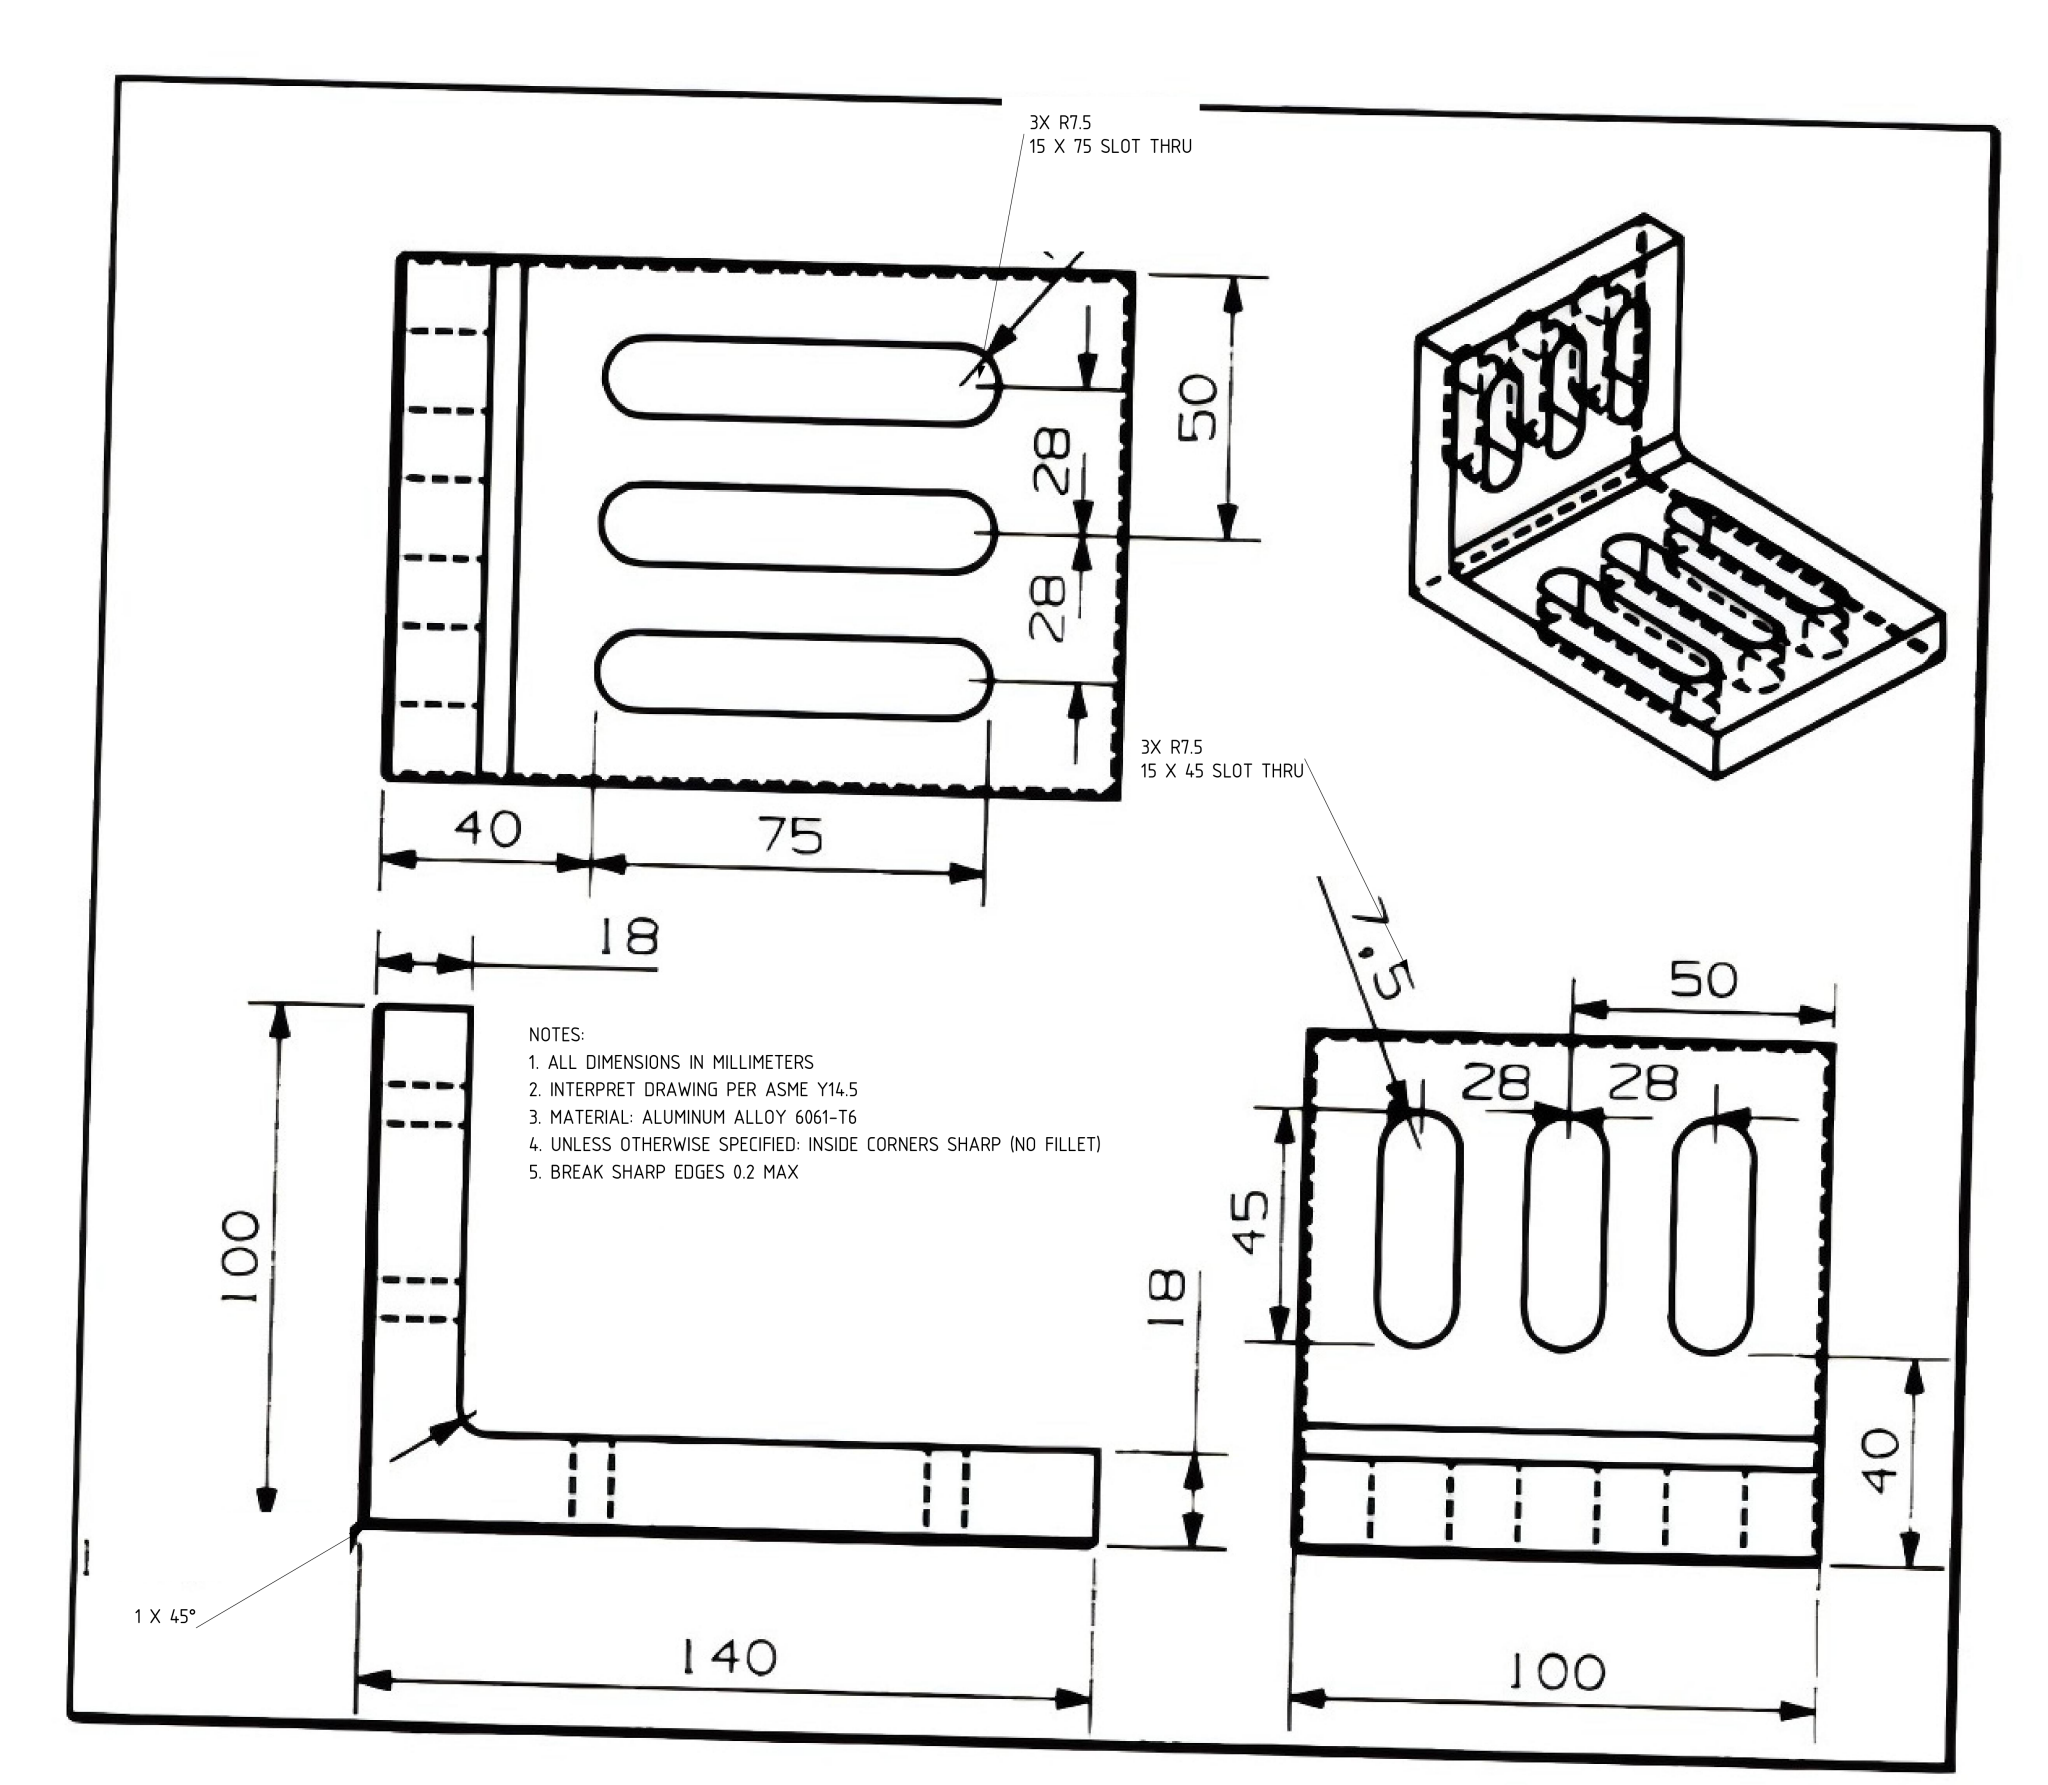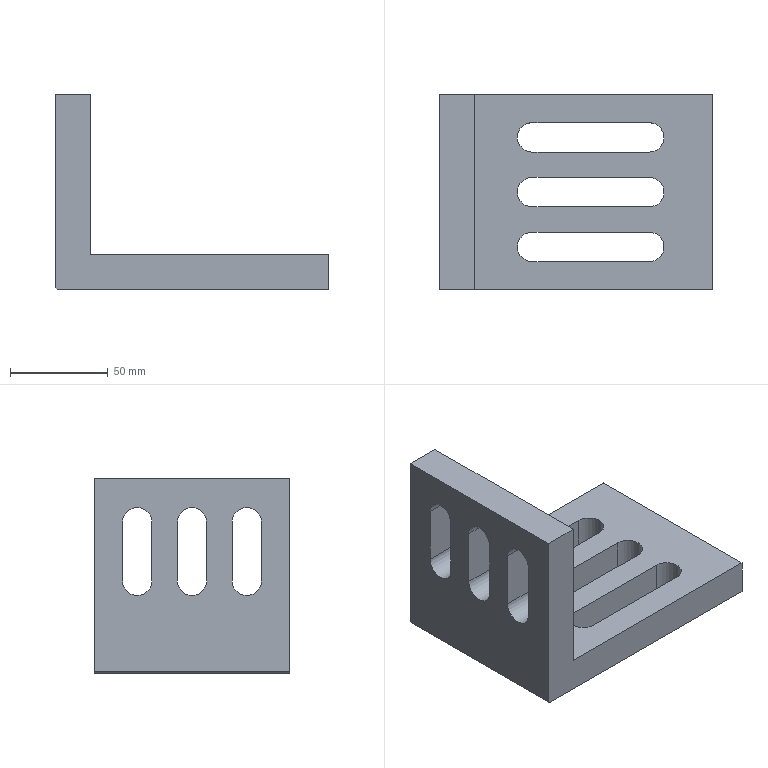Part | NX | mm | 1 solid | 33 faces | box 140 x 100 x 100 mm | volume 307565 mm3 | plane 21 | cylinder 12 | commonest cylinder face diameters 15 x12